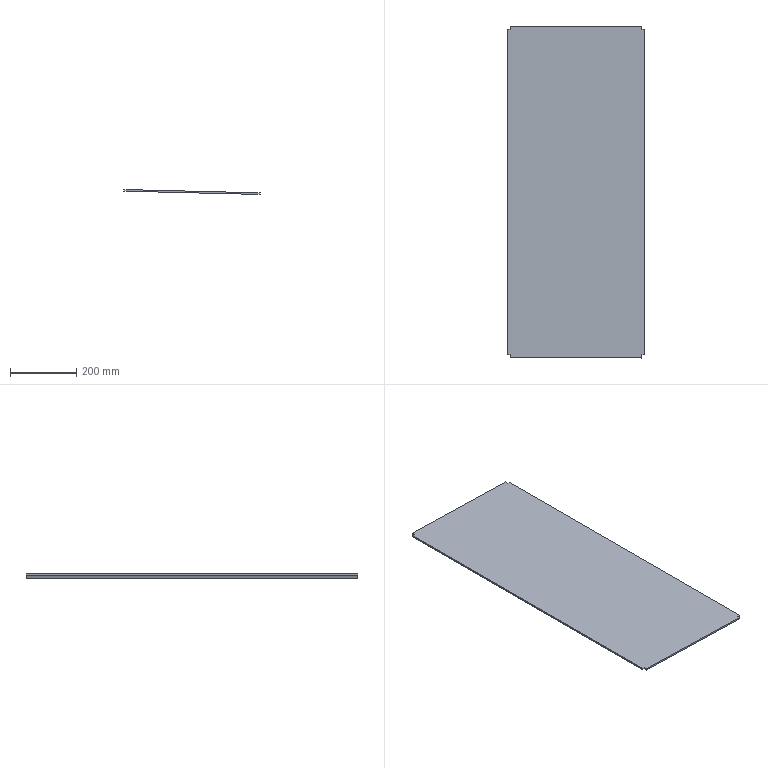Component | SolidWorks | 2012MB0201-1_ASideDoor-1-1_A3004-3 | 1 solid | 14 faces | box 412 x 1001 x 14.85 mm | volume 2060635 mm3 | plane 14
build123d program:
from build123d import *

# Parameters (mm, degrees)
SKETCH1_W               = 412
SKETCH1_H               = 1001
BOSS_EXTRUDE1_DEPTH     = 5
SKETCH2_W               = 7.5
SKETCH2_H               = 9.5
CUT_EXTRUDE2_DEPTH      = 542.259
MIRROR4_COPY_1_SKETCH_W = 7.5
MIRROR4_COPY_1_SKETCH_H = 9.5
MIRROR4_COPY_1_DEPTH    = 542.259


with BuildPart() as part:
    # Sketch1 → Boss-Extrude1 (new body)
    with BuildSketch(Plane(origin=(0, 0, 0), x_dir=(1, 0, 0), z_dir=(0, 1, 0))):
        Rectangle(SKETCH1_W, SKETCH1_H)
    extrude(amount=BOSS_EXTRUDE1_DEPTH)

    # Sketch2 → Cut-Extrude2 (cut, through all)
    with BuildSketch(Plane.XZ):
        with Locations((-202.25, 495.75)):
            Rectangle(SKETCH2_W, SKETCH2_H)
    cut_extrude2 = extrude(amount=-CUT_EXTRUDE2_DEPTH, mode=Mode.SUBTRACT)

    # Mirror3: Cut-Extrude2 across plane
    add(cut_extrude2.mirror(Plane(origin=(0, 0, 0), x_dir=(0, 0, 1), z_dir=(1, 0, 0))), mode=Mode.SUBTRACT)

    # Mirror4: Cut-Extrude2 across plane
    add(cut_extrude2.mirror(Plane.XY), mode=Mode.SUBTRACT)

    # Mirror4 copy 1 sketch → Mirror4 copy 1 (cut, through all)
    with BuildSketch(Plane(origin=(0, 0, 0), x_dir=(-1, 0, 0), z_dir=(0, -1, 0))):
        with Locations((-202.25, 495.75)):
            Rectangle(MIRROR4_COPY_1_SKETCH_W, MIRROR4_COPY_1_SKETCH_H)
    extrude(amount=-MIRROR4_COPY_1_DEPTH, mode=Mode.SUBTRACT)


solid = part.part

# Placed as in the assembly
solid = solid.moved(Location((-1051.304, 481.35, -181.861), (90, 0, 178.629)))
STEP:
#1=CARTESIAN_POINT('',(-49.203,38.282,-6.973));
#2=VERTEX_POINT('',#1);
#3=CARTESIAN_POINT('',(-49.203,38.656,-6.973));
#4=VERTEX_POINT('',#3);
#5=CARTESIAN_POINT('',(-49.203,38.656,-6.973));
#6=DIRECTION('',(-0.,1.,0.));
#7=VECTOR('',#6,39.37);
#8=LINE('',#5,#7);
#9=EDGE_CURVE('',#2,#4,#8,.T.);
#10=ORIENTED_EDGE('',*,*,#9,.F.);
#11=CARTESIAN_POINT('',(-49.498,38.282,-6.966));
#12=VERTEX_POINT('',#11);
#13=CARTESIAN_POINT('',(-49.498,38.282,-6.966));
#14=DIRECTION('',(0.9997,0.,-0.02392));
#15=VECTOR('',#14,39.37);
#16=LINE('',#13,#15);
#17=EDGE_CURVE('',#12,#2,#16,.T.);
#18=ORIENTED_EDGE('',*,*,#17,.F.);
#19=CARTESIAN_POINT('',(-49.498,-0.3799,-6.966));
#20=VERTEX_POINT('',#19);
#21=CARTESIAN_POINT('',(-49.498,38.656,-6.966));
#22=DIRECTION('',(0.,-1.,-0.));
#23=VECTOR('',#22,39.37);
#24=LINE('',#21,#23);
#25=EDGE_CURVE('',#12,#20,#24,.T.);
#26=ORIENTED_EDGE('',*,*,#25,.T.);
#27=CARTESIAN_POINT('',(-49.203,-0.3799,-6.973));
#28=VERTEX_POINT('',#27);
#29=CARTESIAN_POINT('',(-49.498,-0.3799,-6.966));
#30=DIRECTION('',(0.9997,0.,-0.02392));
#31=VECTOR('',#30,39.37);
#32=LINE('',#29,#31);
#33=EDGE_CURVE('',#20,#28,#32,.T.);
#34=ORIENTED_EDGE('',*,*,#33,.T.);
#35=CARTESIAN_POINT('',(-49.203,-0.7539,-6.973));
#36=VERTEX_POINT('',#35);
#37=CARTESIAN_POINT('',(-49.203,-0.7539,-6.973));
#38=DIRECTION('',(0.,-1.,-0.));
#39=VECTOR('',#38,39.37);
#40=LINE('',#37,#39);
#41=EDGE_CURVE('',#28,#36,#40,.T.);
#42=ORIENTED_EDGE('',*,*,#41,.T.);
#43=CARTESIAN_POINT('',(-33.577,-0.7539,-7.347));
#44=VERTEX_POINT('',#43);
#45=CARTESIAN_POINT('',(-49.498,-0.7539,-6.966));
#46=DIRECTION('',(0.9997,0.,-0.02392));
#47=VECTOR('',#46,39.37);
#48=LINE('',#45,#47);
#49=EDGE_CURVE('',#36,#44,#48,.T.);
#50=ORIENTED_EDGE('',*,*,#49,.T.);
#51=CARTESIAN_POINT('',(-33.577,-0.3799,-7.347));
#52=VERTEX_POINT('',#51);
#53=CARTESIAN_POINT('',(-33.577,-0.7539,-7.347));
#54=DIRECTION('',(0.,-1.,-0.));
#55=VECTOR('',#54,39.37);
#56=LINE('',#53,#55);
#57=EDGE_CURVE('',#52,#44,#56,.T.);
#58=ORIENTED_EDGE('',*,*,#57,.F.);
#59=CARTESIAN_POINT('',(-33.282,-0.3799,-7.354));
#60=VERTEX_POINT('',#59);
#61=CARTESIAN_POINT('',(-33.282,-0.3799,-7.354));
#62=DIRECTION('',(-0.9997,-0.,0.02392));
#63=VECTOR('',#62,39.37);
#64=LINE('',#61,#63);
#65=EDGE_CURVE('',#60,#52,#64,.T.);
#66=ORIENTED_EDGE('',*,*,#65,.F.);
#67=CARTESIAN_POINT('',(-33.282,38.282,-7.354));
#68=VERTEX_POINT('',#67);
#69=CARTESIAN_POINT('',(-33.282,38.656,-7.354));
#70=DIRECTION('',(-0.,1.,0.));
#71=VECTOR('',#70,39.37);
#72=LINE('',#69,#71);
#73=EDGE_CURVE('',#60,#68,#72,.T.);
#74=ORIENTED_EDGE('',*,*,#73,.T.);
#75=CARTESIAN_POINT('',(-33.577,38.282,-7.347));
#76=VERTEX_POINT('',#75);
#77=CARTESIAN_POINT('',(-33.282,38.282,-7.354));
#78=DIRECTION('',(-0.9997,-0.,0.02392));
#79=VECTOR('',#78,39.37);
#80=LINE('',#77,#79);
#81=EDGE_CURVE('',#68,#76,#80,.T.);
#82=ORIENTED_EDGE('',*,*,#81,.T.);
#83=CARTESIAN_POINT('',(-33.577,38.656,-7.347));
#84=VERTEX_POINT('',#83);
#85=CARTESIAN_POINT('',(-33.577,38.656,-7.347));
#86=DIRECTION('',(-0.,1.,0.));
#87=VECTOR('',#86,39.37);
#88=LINE('',#85,#87);
#89=EDGE_CURVE('',#76,#84,#88,.T.);
#90=ORIENTED_EDGE('',*,*,#89,.T.);
#91=CARTESIAN_POINT('',(-49.498,38.656,-6.966));
#92=DIRECTION('',(-0.9997,-0.,0.02392));
#93=VECTOR('',#92,39.37);
#94=LINE('',#91,#93);
#95=EDGE_CURVE('',#84,#4,#94,.T.);
#96=ORIENTED_EDGE('',*,*,#95,.T.);
#97=EDGE_LOOP('',(#10,#18,#26,#34,#42,#50,#58,#66,#74,#82,#90,#96));
#98=FACE_OUTER_BOUND('',#97,.T.);
#99=CARTESIAN_POINT('',(-41.39,18.951,-7.16));
#100=DIRECTION('',(0.02392,0.,0.9997));
#101=DIRECTION('',(0.,-1.,-0.));
#102=AXIS2_PLACEMENT_3D('',#99,#100,#101);
#103=PLANE('',#102);
#104=ADVANCED_FACE('',(#98),#103,.T.);
#105=CARTESIAN_POINT('',(-49.503,38.282,-7.163));
#106=VERTEX_POINT('',#105);
#107=CARTESIAN_POINT('',(-49.207,38.282,-7.17));
#108=VERTEX_POINT('',#107);
#109=CARTESIAN_POINT('',(-49.503,38.282,-7.163));
#110=DIRECTION('',(0.9997,0.,-0.02392));
#111=VECTOR('',#110,39.37);
#112=LINE('',#109,#111);
#113=EDGE_CURVE('',#106,#108,#112,.T.);
#114=ORIENTED_EDGE('',*,*,#113,.T.);
#115=CARTESIAN_POINT('',(-49.207,38.656,-7.17));
#116=VERTEX_POINT('',#115);
#117=CARTESIAN_POINT('',(-49.207,38.656,-7.17));
#118=DIRECTION('',(-0.,1.,0.));
#119=VECTOR('',#118,39.37);
#120=LINE('',#117,#119);
#121=EDGE_CURVE('',#108,#116,#120,.T.);
#122=ORIENTED_EDGE('',*,*,#121,.T.);
#123=CARTESIAN_POINT('',(-33.582,38.656,-7.544));
#124=VERTEX_POINT('',#123);
#125=CARTESIAN_POINT('',(-49.503,38.656,-7.163));
#126=DIRECTION('',(-0.9997,-0.,0.02392));
#127=VECTOR('',#126,39.37);
#128=LINE('',#125,#127);
#129=EDGE_CURVE('',#124,#116,#128,.T.);
#130=ORIENTED_EDGE('',*,*,#129,.F.);
#131=CARTESIAN_POINT('',(-33.582,38.282,-7.544));
#132=VERTEX_POINT('',#131);
#133=CARTESIAN_POINT('',(-33.582,38.656,-7.544));
#134=DIRECTION('',(-0.,1.,0.));
#135=VECTOR('',#134,39.37);
#136=LINE('',#133,#135);
#137=EDGE_CURVE('',#132,#124,#136,.T.);
#138=ORIENTED_EDGE('',*,*,#137,.F.);
#139=CARTESIAN_POINT('',(-33.287,38.282,-7.551));
#140=VERTEX_POINT('',#139);
#141=CARTESIAN_POINT('',(-33.287,38.282,-7.551));
#142=DIRECTION('',(-0.9997,-0.,0.02392));
#143=VECTOR('',#142,39.37);
#144=LINE('',#141,#143);
#145=EDGE_CURVE('',#140,#132,#144,.T.);
#146=ORIENTED_EDGE('',*,*,#145,.F.);
#147=CARTESIAN_POINT('',(-33.287,-0.3799,-7.551));
#148=VERTEX_POINT('',#147);
#149=CARTESIAN_POINT('',(-33.287,38.656,-7.551));
#150=DIRECTION('',(-0.,1.,0.));
#151=VECTOR('',#150,39.37);
#152=LINE('',#149,#151);
#153=EDGE_CURVE('',#148,#140,#152,.T.);
#154=ORIENTED_EDGE('',*,*,#153,.F.);
#155=CARTESIAN_POINT('',(-33.582,-0.3799,-7.544));
#156=VERTEX_POINT('',#155);
#157=CARTESIAN_POINT('',(-33.287,-0.3799,-7.551));
#158=DIRECTION('',(-0.9997,-0.,0.02392));
#159=VECTOR('',#158,39.37);
#160=LINE('',#157,#159);
#161=EDGE_CURVE('',#148,#156,#160,.T.);
#162=ORIENTED_EDGE('',*,*,#161,.T.);
#163=CARTESIAN_POINT('',(-33.582,-0.7539,-7.544));
#164=VERTEX_POINT('',#163);
#165=CARTESIAN_POINT('',(-33.582,-0.7539,-7.544));
#166=DIRECTION('',(0.,-1.,-0.));
#167=VECTOR('',#166,39.37);
#168=LINE('',#165,#167);
#169=EDGE_CURVE('',#156,#164,#168,.T.);
#170=ORIENTED_EDGE('',*,*,#169,.T.);
#171=CARTESIAN_POINT('',(-49.207,-0.7539,-7.17));
#172=VERTEX_POINT('',#171);
#173=CARTESIAN_POINT('',(-49.503,-0.7539,-7.163));
#174=DIRECTION('',(0.9997,0.,-0.02392));
#175=VECTOR('',#174,39.37);
#176=LINE('',#173,#175);
#177=EDGE_CURVE('',#172,#164,#176,.T.);
#178=ORIENTED_EDGE('',*,*,#177,.F.);
#179=CARTESIAN_POINT('',(-49.207,-0.3799,-7.17));
#180=VERTEX_POINT('',#179);
#181=CARTESIAN_POINT('',(-49.207,-0.7539,-7.17));
#182=DIRECTION('',(0.,-1.,-0.));
#183=VECTOR('',#182,39.37);
#184=LINE('',#181,#183);
#185=EDGE_CURVE('',#180,#172,#184,.T.);
#186=ORIENTED_EDGE('',*,*,#185,.F.);
#187=CARTESIAN_POINT('',(-49.503,-0.3799,-7.163));
#188=VERTEX_POINT('',#187);
#189=CARTESIAN_POINT('',(-49.503,-0.3799,-7.163));
#190=DIRECTION('',(0.9997,0.,-0.02392));
#191=VECTOR('',#190,39.37);
#192=LINE('',#189,#191);
#193=EDGE_CURVE('',#188,#180,#192,.T.);
#194=ORIENTED_EDGE('',*,*,#193,.F.);
#195=CARTESIAN_POINT('',(-49.503,38.656,-7.163));
#196=DIRECTION('',(0.,-1.,-0.));
#197=VECTOR('',#196,39.37);
#198=LINE('',#195,#197);
#199=EDGE_CURVE('',#106,#188,#198,.T.);
#200=ORIENTED_EDGE('',*,*,#199,.F.);
#201=EDGE_LOOP('',(#114,#122,#130,#138,#146,#154,#162,#170,#178,#186,#194,#200));
#202=FACE_OUTER_BOUND('',#201,.T.);
#203=CARTESIAN_POINT('',(-41.395,18.951,-7.357));
#204=DIRECTION('',(0.02392,0.,0.9997));
#205=DIRECTION('',(0.,-1.,-0.));
#206=AXIS2_PLACEMENT_3D('',#203,#204,#205);
#207=PLANE('',#206);
#208=ADVANCED_FACE('',(#202),#207,.F.);
#209=CARTESIAN_POINT('',(-49.203,38.656,-6.973));
#210=DIRECTION('',(-0.02392,-0.,-0.9997));
#211=VECTOR('',#210,39.37);
#212=LINE('',#209,#211);
#213=EDGE_CURVE('',#4,#116,#212,.T.);
#214=ORIENTED_EDGE('',*,*,#213,.F.);
#215=ORIENTED_EDGE('',*,*,#95,.F.);
#216=CARTESIAN_POINT('',(-33.577,38.656,-7.347));
#217=DIRECTION('',(-0.02392,-0.,-0.9997));
#218=VECTOR('',#217,39.37);
#219=LINE('',#216,#218);
#220=EDGE_CURVE('',#84,#124,#219,.T.);
#221=ORIENTED_EDGE('',*,*,#220,.T.);
#222=ORIENTED_EDGE('',*,*,#129,.T.);
#223=EDGE_LOOP('',(#214,#215,#221,#222));
#224=FACE_OUTER_BOUND('',#223,.T.);
#225=CARTESIAN_POINT('',(-49.498,38.656,-6.966));
#226=DIRECTION('',(0.,-1.,-0.));
#227=DIRECTION('',(0.9997,0.,-0.02392));
#228=AXIS2_PLACEMENT_3D('',#225,#226,#227);
#229=PLANE('',#228);
#230=ADVANCED_FACE('',(#224),#229,.F.);
#231=CARTESIAN_POINT('',(-49.498,38.282,-6.966));
#232=DIRECTION('',(-0.02392,-0.,-0.9997));
#233=VECTOR('',#232,39.37);
#234=LINE('',#231,#233);
#235=EDGE_CURVE('',#12,#106,#234,.T.);
#236=ORIENTED_EDGE('',*,*,#235,.T.);
#237=ORIENTED_EDGE('',*,*,#199,.T.);
#238=CARTESIAN_POINT('',(-49.498,-0.3799,-6.966));
#239=DIRECTION('',(-0.02392,-0.,-0.9997));
#240=VECTOR('',#239,39.37);
#241=LINE('',#238,#240);
#242=EDGE_CURVE('',#20,#188,#241,.T.);
#243=ORIENTED_EDGE('',*,*,#242,.F.);
#244=ORIENTED_EDGE('',*,*,#25,.F.);
#245=EDGE_LOOP('',(#236,#237,#243,#244));
#246=FACE_OUTER_BOUND('',#245,.T.);
#247=CARTESIAN_POINT('',(-49.498,38.656,-6.966));
#248=DIRECTION('',(0.9997,0.,-0.02392));
#249=DIRECTION('',(-0.,1.,0.));
#250=AXIS2_PLACEMENT_3D('',#247,#248,#249);
#251=PLANE('',#250);
#252=ADVANCED_FACE('',(#246),#251,.F.);
#253=ORIENTED_EDGE('',*,*,#153,.T.);
#254=CARTESIAN_POINT('',(-33.282,38.282,-7.354));
#255=DIRECTION('',(-0.02392,-0.,-0.9997));
#256=VECTOR('',#255,39.37);
#257=LINE('',#254,#256);
#258=EDGE_CURVE('',#68,#140,#257,.T.);
#259=ORIENTED_EDGE('',*,*,#258,.F.);
#260=ORIENTED_EDGE('',*,*,#73,.F.);
#261=CARTESIAN_POINT('',(-33.282,-0.3799,-7.354));
#262=DIRECTION('',(-0.02392,-0.,-0.9997));
#263=VECTOR('',#262,39.37);
#264=LINE('',#261,#263);
#265=EDGE_CURVE('',#60,#148,#264,.T.);
#266=ORIENTED_EDGE('',*,*,#265,.T.);
#267=EDGE_LOOP('',(#253,#259,#260,#266));
#268=FACE_OUTER_BOUND('',#267,.T.);
#269=CARTESIAN_POINT('',(-33.282,38.656,-7.354));
#270=DIRECTION('',(-0.9997,-0.,0.02392));
#271=DIRECTION('',(0.,-1.,-0.));
#272=AXIS2_PLACEMENT_3D('',#269,#270,#271);
#273=PLANE('',#272);
#274=ADVANCED_FACE('',(#268),#273,.F.);
#275=CARTESIAN_POINT('',(-33.577,-0.7539,-7.347));
#276=DIRECTION('',(-0.02392,-0.,-0.9997));
#277=VECTOR('',#276,39.37);
#278=LINE('',#275,#277);
#279=EDGE_CURVE('',#44,#164,#278,.T.);
#280=ORIENTED_EDGE('',*,*,#279,.F.);
#281=ORIENTED_EDGE('',*,*,#49,.F.);
#282=CARTESIAN_POINT('',(-49.203,-0.7539,-6.973));
#283=DIRECTION('',(-0.02392,-0.,-0.9997));
#284=VECTOR('',#283,39.37);
#285=LINE('',#282,#284);
#286=EDGE_CURVE('',#36,#172,#285,.T.);
#287=ORIENTED_EDGE('',*,*,#286,.T.);
#288=ORIENTED_EDGE('',*,*,#177,.T.);
#289=EDGE_LOOP('',(#280,#281,#287,#288));
#290=FACE_OUTER_BOUND('',#289,.T.);
#291=CARTESIAN_POINT('',(-49.498,-0.7539,-6.966));
#292=DIRECTION('',(-0.,1.,0.));
#293=DIRECTION('',(-0.9997,-0.,0.02392));
#294=AXIS2_PLACEMENT_3D('',#291,#292,#293);
#295=PLANE('',#294);
#296=ADVANCED_FACE('',(#290),#295,.F.);
#297=ORIENTED_EDGE('',*,*,#185,.T.);
#298=ORIENTED_EDGE('',*,*,#286,.F.);
#299=ORIENTED_EDGE('',*,*,#41,.F.);
#300=CARTESIAN_POINT('',(-49.203,-0.3799,-6.973));
#301=DIRECTION('',(-0.02392,-0.,-0.9997));
#302=VECTOR('',#301,39.37);
#303=LINE('',#300,#302);
#304=EDGE_CURVE('',#28,#180,#303,.T.);
#305=ORIENTED_EDGE('',*,*,#304,.T.);
#306=EDGE_LOOP('',(#297,#298,#299,#305));
#307=FACE_OUTER_BOUND('',#306,.T.);
#308=CARTESIAN_POINT('',(-49.203,-0.7539,-6.973));
#309=DIRECTION('',(0.9997,0.,-0.02392));
#310=DIRECTION('',(-0.,1.,0.));
#311=AXIS2_PLACEMENT_3D('',#308,#309,#310);
#312=PLANE('',#311);
#313=ADVANCED_FACE('',(#307),#312,.F.);
#314=ORIENTED_EDGE('',*,*,#193,.T.);
#315=ORIENTED_EDGE('',*,*,#304,.F.);
#316=ORIENTED_EDGE('',*,*,#33,.F.);
#317=ORIENTED_EDGE('',*,*,#242,.T.);
#318=EDGE_LOOP('',(#314,#315,#316,#317));
#319=FACE_OUTER_BOUND('',#318,.T.);
#320=CARTESIAN_POINT('',(-49.498,-0.3799,-6.966));
#321=DIRECTION('',(-0.,1.,0.));
#322=DIRECTION('',(-0.9997,-0.,0.02392));
#323=AXIS2_PLACEMENT_3D('',#320,#321,#322);
#324=PLANE('',#323);
#325=ADVANCED_FACE('',(#319),#324,.F.);
#326=ORIENTED_EDGE('',*,*,#161,.F.);
#327=ORIENTED_EDGE('',*,*,#265,.F.);
#328=ORIENTED_EDGE('',*,*,#65,.T.);
#329=CARTESIAN_POINT('',(-33.577,-0.3799,-7.347));
#330=DIRECTION('',(-0.02392,-0.,-0.9997));
#331=VECTOR('',#330,39.37);
#332=LINE('',#329,#331);
#333=EDGE_CURVE('',#52,#156,#332,.T.);
#334=ORIENTED_EDGE('',*,*,#333,.T.);
#335=EDGE_LOOP('',(#326,#327,#328,#334));
#336=FACE_OUTER_BOUND('',#335,.T.);
#337=CARTESIAN_POINT('',(-33.282,-0.3799,-7.354));
#338=DIRECTION('',(0.,-1.,-0.));
#339=DIRECTION('',(0.9997,0.,-0.02392));
#340=AXIS2_PLACEMENT_3D('',#337,#338,#339);
#341=PLANE('',#340);
#342=ADVANCED_FACE('',(#336),#341,.T.);
#343=ORIENTED_EDGE('',*,*,#169,.F.);
#344=ORIENTED_EDGE('',*,*,#333,.F.);
#345=ORIENTED_EDGE('',*,*,#57,.T.);
#346=ORIENTED_EDGE('',*,*,#279,.T.);
#347=EDGE_LOOP('',(#343,#344,#345,#346));
#348=FACE_OUTER_BOUND('',#347,.T.);
#349=CARTESIAN_POINT('',(-33.577,-0.7539,-7.347));
#350=DIRECTION('',(0.9997,0.,-0.02392));
#351=DIRECTION('',(-0.,1.,0.));
#352=AXIS2_PLACEMENT_3D('',#349,#350,#351);
#353=PLANE('',#352);
#354=ADVANCED_FACE('',(#348),#353,.T.);
#355=ORIENTED_EDGE('',*,*,#137,.T.);
#356=ORIENTED_EDGE('',*,*,#220,.F.);
#357=ORIENTED_EDGE('',*,*,#89,.F.);
#358=CARTESIAN_POINT('',(-33.577,38.282,-7.347));
#359=DIRECTION('',(-0.02392,-0.,-0.9997));
#360=VECTOR('',#359,39.37);
#361=LINE('',#358,#360);
#362=EDGE_CURVE('',#76,#132,#361,.T.);
#363=ORIENTED_EDGE('',*,*,#362,.T.);
#364=EDGE_LOOP('',(#355,#356,#357,#363));
#365=FACE_OUTER_BOUND('',#364,.T.);
#366=CARTESIAN_POINT('',(-33.577,38.656,-7.347));
#367=DIRECTION('',(-0.9997,-0.,0.02392));
#368=DIRECTION('',(0.,-1.,-0.));
#369=AXIS2_PLACEMENT_3D('',#366,#367,#368);
#370=PLANE('',#369);
#371=ADVANCED_FACE('',(#365),#370,.F.);
#372=ORIENTED_EDGE('',*,*,#145,.T.);
#373=ORIENTED_EDGE('',*,*,#362,.F.);
#374=ORIENTED_EDGE('',*,*,#81,.F.);
#375=ORIENTED_EDGE('',*,*,#258,.T.);
#376=EDGE_LOOP('',(#372,#373,#374,#375));
#377=FACE_OUTER_BOUND('',#376,.T.);
#378=CARTESIAN_POINT('',(-33.282,38.282,-7.354));
#379=DIRECTION('',(0.,-1.,-0.));
#380=DIRECTION('',(0.9997,0.,-0.02392));
#381=AXIS2_PLACEMENT_3D('',#378,#379,#380);
#382=PLANE('',#381);
#383=ADVANCED_FACE('',(#377),#382,.F.);
#384=ORIENTED_EDGE('',*,*,#113,.F.);
#385=ORIENTED_EDGE('',*,*,#235,.F.);
#386=ORIENTED_EDGE('',*,*,#17,.T.);
#387=CARTESIAN_POINT('',(-49.203,38.282,-6.973));
#388=DIRECTION('',(-0.02392,-0.,-0.9997));
#389=VECTOR('',#388,39.37);
#390=LINE('',#387,#389);
#391=EDGE_CURVE('',#2,#108,#390,.T.);
#392=ORIENTED_EDGE('',*,*,#391,.T.);
#393=EDGE_LOOP('',(#384,#385,#386,#392));
#394=FACE_OUTER_BOUND('',#393,.T.);
#395=CARTESIAN_POINT('',(-49.498,38.282,-6.966));
#396=DIRECTION('',(-0.,1.,0.));
#397=DIRECTION('',(-0.9997,-0.,0.02392));
#398=AXIS2_PLACEMENT_3D('',#395,#396,#397);
#399=PLANE('',#398);
#400=ADVANCED_FACE('',(#394),#399,.T.);
#401=ORIENTED_EDGE('',*,*,#121,.F.);
#402=ORIENTED_EDGE('',*,*,#391,.F.);
#403=ORIENTED_EDGE('',*,*,#9,.T.);
#404=ORIENTED_EDGE('',*,*,#213,.T.);
#405=EDGE_LOOP('',(#401,#402,#403,#404));
#406=FACE_OUTER_BOUND('',#405,.T.);
#407=CARTESIAN_POINT('',(-49.203,38.656,-6.973));
#408=DIRECTION('',(-0.9997,-0.,0.02392));
#409=DIRECTION('',(0.,-1.,-0.));
#410=AXIS2_PLACEMENT_3D('',#407,#408,#409);
#411=PLANE('',#410);
#412=ADVANCED_FACE('',(#406),#411,.T.);
#413=CLOSED_SHELL('',(#104,#208,#230,#252,#274,#296,#313,#325,#342,#354,#371,#383,#400,#412));
#414=MANIFOLD_SOLID_BREP('',#413);
#415=CARTESIAN_POINT('',(0.,0.,0.));
#416=DIRECTION('',(0.,0.,1.));
#417=DIRECTION('',(1.,0.,0.));
#418=AXIS2_PLACEMENT_3D('',#415,#416,#417);
#419=(LENGTH_UNIT()NAMED_UNIT(*)SI_UNIT($,.METRE.));
#420=LENGTH_MEASURE_WITH_UNIT(LENGTH_MEASURE(0.0254),#419);
#421=DIMENSIONAL_EXPONENTS(1.,0.,0.,0.,0.,0.,0.);
#422=(CONVERSION_BASED_UNIT('',#420)LENGTH_UNIT()NAMED_UNIT(#421));
#423=UNCERTAINTY_MEASURE_WITH_UNIT(LENGTH_MEASURE(0.00001),#422,'','');
#424=(NAMED_UNIT(*)PLANE_ANGLE_UNIT()SI_UNIT($,.RADIAN.));
#425=(NAMED_UNIT(*)SI_UNIT($,.STERADIAN.)SOLID_ANGLE_UNIT());
#426=(GEOMETRIC_REPRESENTATION_CONTEXT(3)GLOBAL_UNCERTAINTY_ASSIGNED_CONTEXT((#423))GLOBAL_UNIT_ASSIGNED_CONTEXT((#422,#424,#425))REPRESENTATION_CONTEXT('',''));
#427=ADVANCED_BREP_SHAPE_REPRESENTATION('',(#414,#418),#426);
#428=COLOUR_RGB('',0.7922,0.8196,0.9333);
#429=FILL_AREA_STYLE_COLOUR('',#428);
#430=FILL_AREA_STYLE('',(#429));
#431=SURFACE_STYLE_FILL_AREA(#430);
#432=SURFACE_SIDE_STYLE('',(#431));
#433=SURFACE_STYLE_USAGE(.BOTH.,#432);
#434=PRESENTATION_STYLE_ASSIGNMENT((#433));
#435=STYLED_ITEM('',(#434),#414);
#436=PRESENTATION_LAYER_ASSIGNMENT('','',(#435));
#437=(LENGTH_UNIT()NAMED_UNIT(*)SI_UNIT($,.METRE.));
#438=LENGTH_MEASURE_WITH_UNIT(LENGTH_MEASURE(0.0254),#437);
#439=DIMENSIONAL_EXPONENTS(1.,0.,0.,0.,0.,0.,0.);
#440=(CONVERSION_BASED_UNIT('',#438)LENGTH_UNIT()NAMED_UNIT(#439));
#441=UNCERTAINTY_MEASURE_WITH_UNIT(LENGTH_MEASURE(0.00001),#440,'','');
#442=(NAMED_UNIT(*)PLANE_ANGLE_UNIT()SI_UNIT($,.RADIAN.));
#443=(NAMED_UNIT(*)SI_UNIT($,.STERADIAN.)SOLID_ANGLE_UNIT());
#444=(GEOMETRIC_REPRESENTATION_CONTEXT(3)GLOBAL_UNCERTAINTY_ASSIGNED_CONTEXT((#441))GLOBAL_UNIT_ASSIGNED_CONTEXT((#440,#442,#443))REPRESENTATION_CONTEXT('',''));
#445=MECHANICAL_DESIGN_GEOMETRIC_PRESENTATION_REPRESENTATION('',(#435),#444);